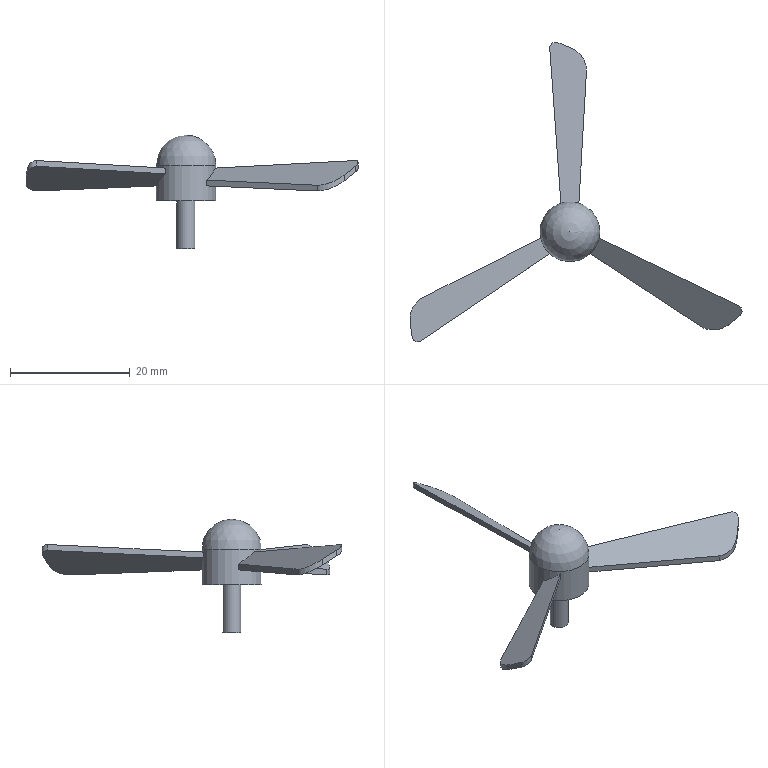Component | NX | PROPELLER_2 | 5 solids | 30 faces | volume 1137 mm3 | plane 18 | cylinder 11 | sphere 1 | commonest cylinder face diameters 10 x4 8 x3 2 x3 3 x1